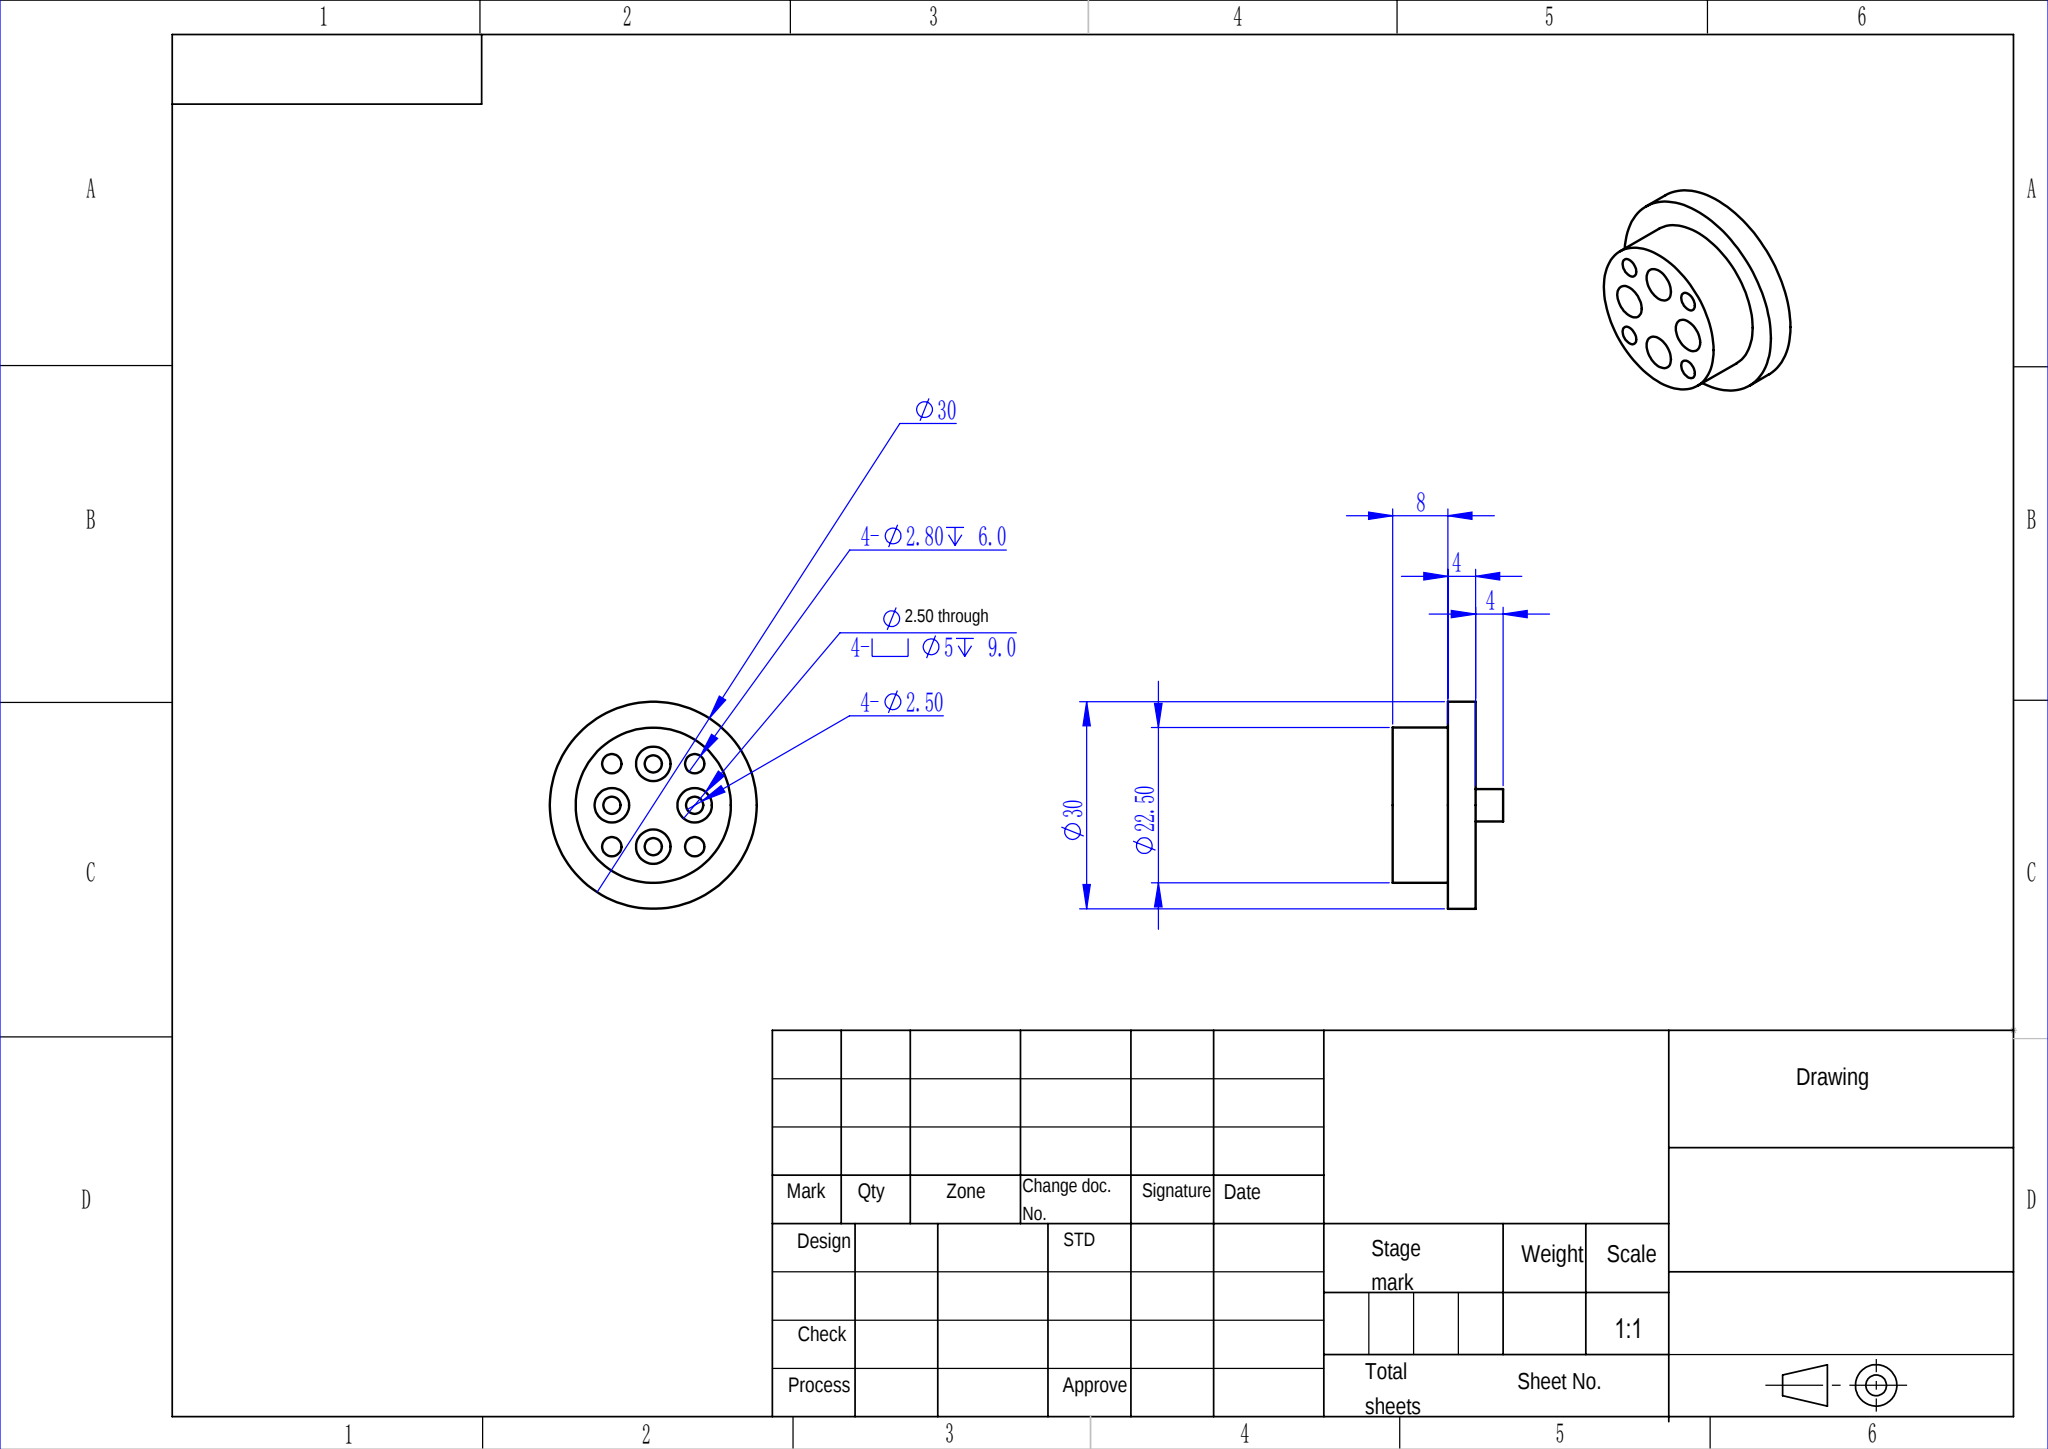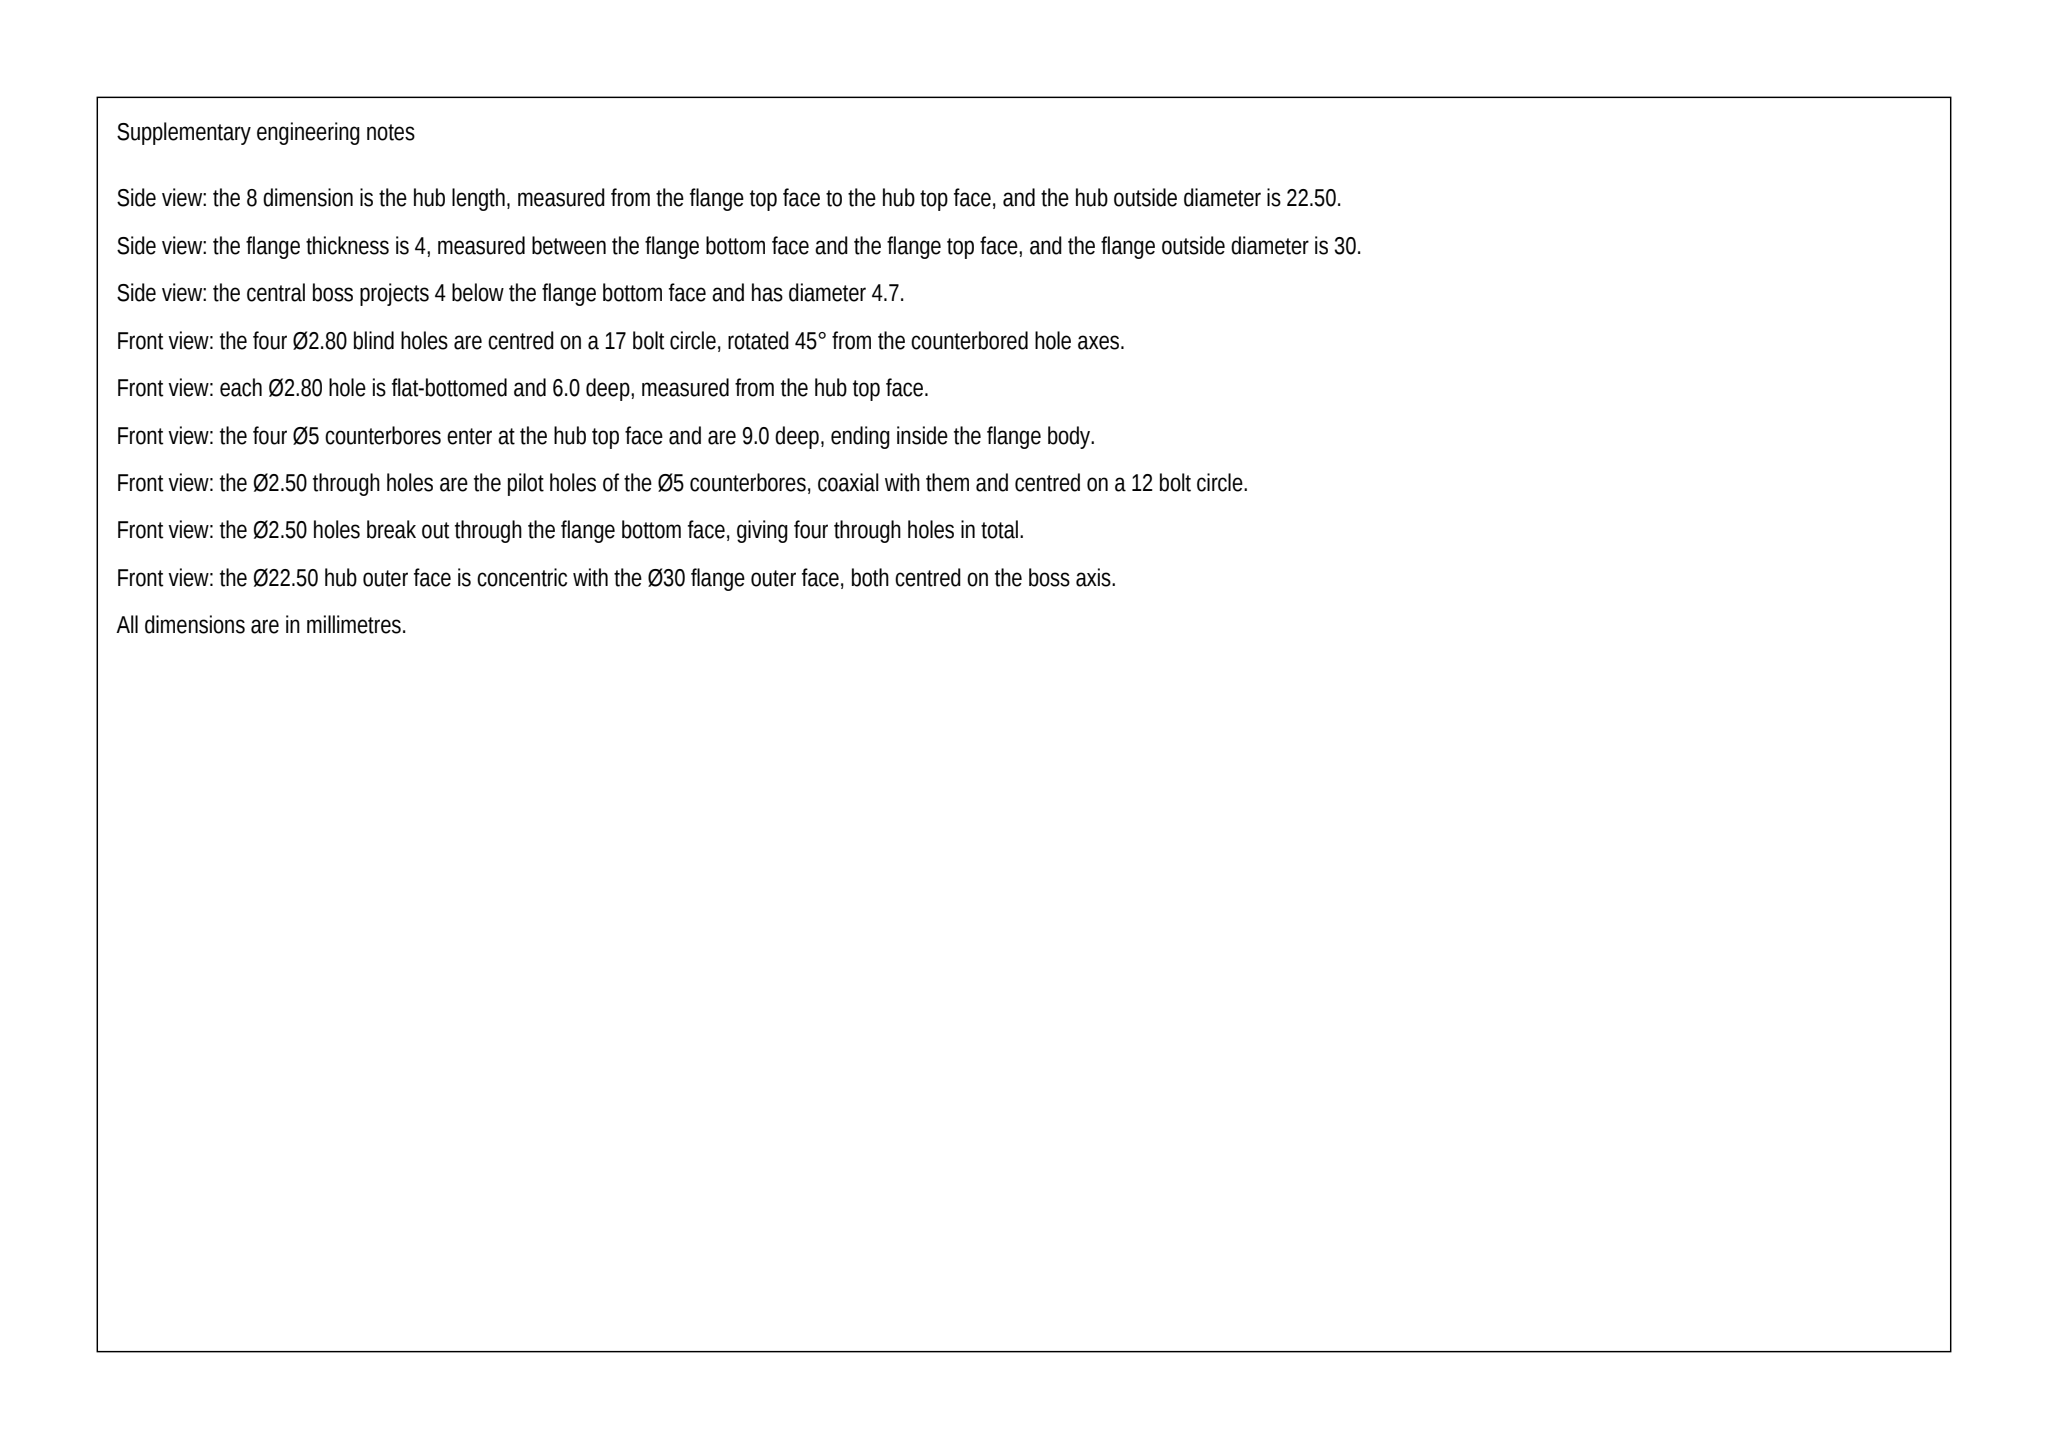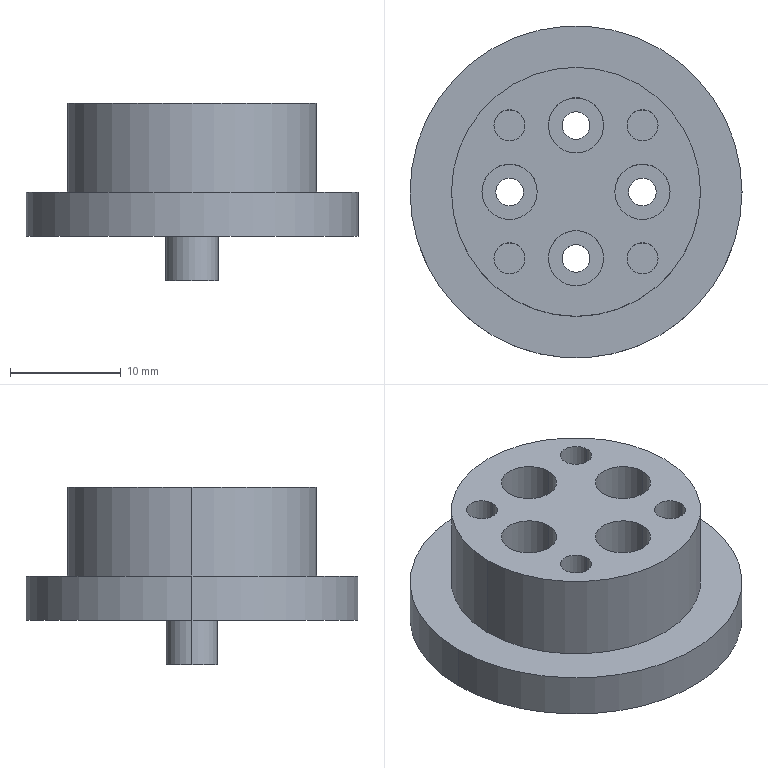Part | SolidWorks | mm | 1 solid | 42 faces | box 30 x 30 x 16 mm | volume 5164 mm3 | cylinder 30 | plane 12 | commonest cylinder face diameters 2.8 x8 5 x8 2.5 x8 22.5 x2 4.7 x2 30 x2
Drawing notes:
4X Ø2.50 THRU CBORE Ø5 DP 9.0 EQ SP ON Ø12 B.C., HOLES ON CL | from the solid: Ø2.5 bores at (15,21),(15,9),(21,15),(9,15) z4-7; Ø5 c'bores same axes z7-16; part axis (15,15) -> R6 = Ø12 B.C., 90 deg spacing on X/Y centerlines
BACK FACE BOSS: Ø4.7 x 4 LG, COAX W/ Ø30 | from the solid: cylinder boss/shaft dia 4.7, axis z at (15,15), from 0.0 to 4.0
4X Ø2.80 DP 6.0 ON Ø16.97 B.C. | from the solid: 4x dia 2.8 holes at (21,21),(21,9),(9,21),(9,9) = R8.485 from axis (15,15)
4X Ø2.80 HOLES EQ SP 90° APART, AT 45° TO CL | from the solid: hole centers offset ±6,±6 from axis -> 45°,135°,225°,315°, equally spaced
build123d program:
from build123d import *

# Parameters (mm, degrees)
SKETCH1_R           = 15
SKETCH1_R_2         = 1.25
BOSS_EXTRUDE1_DEPTH = 4
SKETCH2_R           = 2.35
BOSS_EXTRUDE2_DEPTH = 4
SKETCH3_R           = 11.25
BOSS_EXTRUDE3_DEPTH = 8
CUT_EXTRUDE2_START  = -15
SKETCH4_R           = 1.25
CUT_EXTRUDE2_DEPTH  = 15
SKETCH5_R           = 2.5
CUT_EXTRUDE3_DEPTH  = 9
SKETCH6_R           = 1.4
CUT_EXTRUDE4_DEPTH  = 6


with BuildPart() as part:
    # Sketch1 → Boss-Extrude1 (new body)
    with BuildSketch(Plane.XY):
        Circle(SKETCH1_R)
        with Locations((0, 6)):
            Circle(SKETCH1_R_2, mode=Mode.SUBTRACT)
        with Locations((6, 0)):
            Circle(SKETCH1_R_2, mode=Mode.SUBTRACT)
        with Locations((0, -6)):
            Circle(SKETCH1_R_2, mode=Mode.SUBTRACT)
        with Locations((-6, 0)):
            Circle(SKETCH1_R_2, mode=Mode.SUBTRACT)
    extrude(amount=BOSS_EXTRUDE1_DEPTH)

    # Sketch2 → Boss-Extrude2 (add)
    with BuildSketch(Plane(origin=(0, 0, 0), x_dir=(-1, 0, 0), z_dir=(0, 0, -1))):
        Circle(SKETCH2_R)
    extrude(amount=BOSS_EXTRUDE2_DEPTH)

    # Sketch3 → Boss-Extrude3 (add)
    with BuildSketch(Plane.XY.offset(4)):
        Circle(SKETCH3_R)
    extrude(amount=BOSS_EXTRUDE3_DEPTH)

    # Sketch4 → Cut-Extrude2 (cut)
    with BuildSketch(Plane.XY.offset(12).offset(CUT_EXTRUDE2_START)):
        with Locations((0, -6)):
            Circle(SKETCH4_R)
        with Locations((6, 0)):
            Circle(SKETCH4_R)
        with Locations((0, 6)):
            Circle(SKETCH4_R)
        with Locations((-6, 0)):
            Circle(SKETCH4_R)
    extrude(amount=CUT_EXTRUDE2_DEPTH, mode=Mode.SUBTRACT)

    # Sketch5 → Cut-Extrude3 (cut)
    with BuildSketch(Plane.XY.offset(12)):
        with Locations((0, 6)):
            Circle(SKETCH5_R)
        with Locations((6, 0)):
            Circle(SKETCH5_R)
        with Locations((0, -6)):
            Circle(SKETCH5_R)
        with Locations((-6, 0)):
            Circle(SKETCH5_R)
    extrude(amount=-CUT_EXTRUDE3_DEPTH, mode=Mode.SUBTRACT)

    # Sketch6 → Cut-Extrude4 (cut)
    with BuildSketch(Plane.XY.offset(12)):
        with Locations((6.01, 6.01)):
            Circle(SKETCH6_R)
        with Locations((6.01, -6.01)):
            Circle(SKETCH6_R)
        with Locations((-6.01, -6.01)):
            Circle(SKETCH6_R)
        with Locations((-6.01, 6.01)):
            Circle(SKETCH6_R)
    extrude(amount=-CUT_EXTRUDE4_DEPTH, mode=Mode.SUBTRACT)


solid = part.part